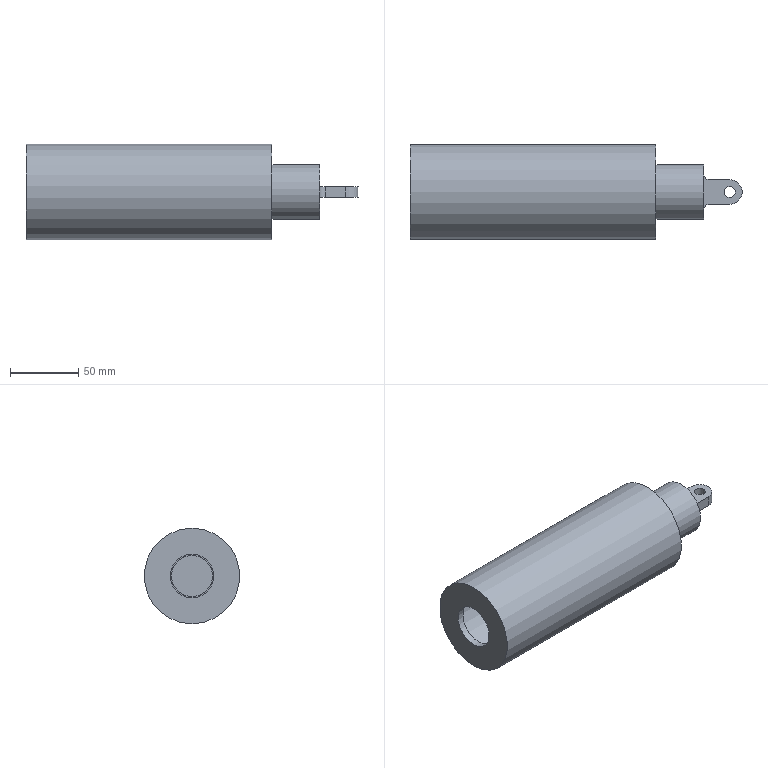Component | NX | OUTER_TUBE | 2 solids | 20 faces | volume 230685 mm3 | plane 11 | cylinder 9 | commonest cylinder face diameters 8 x3 18 x1 32 x1 60 x1 30 x1 40 x1 70 x1